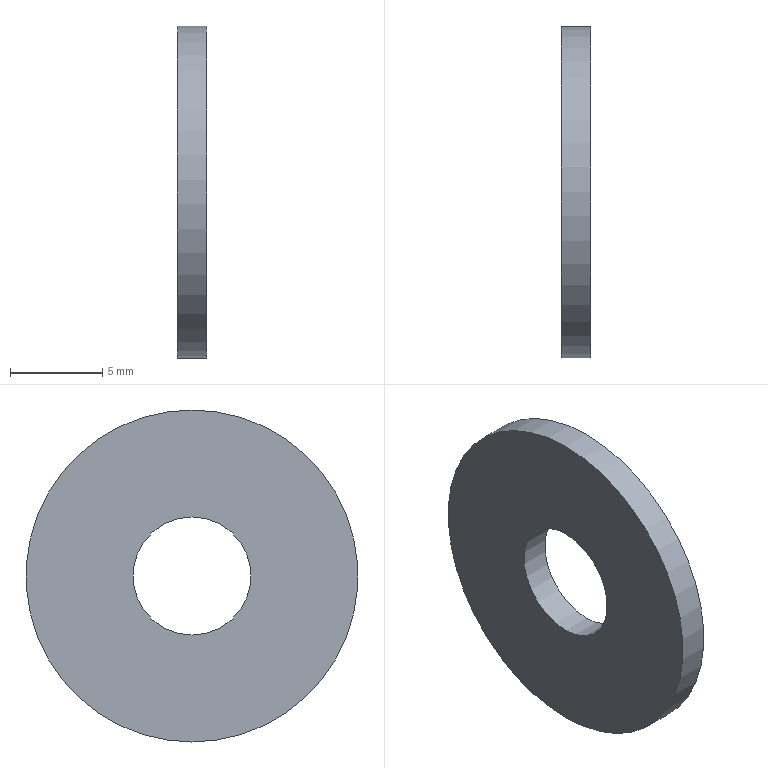Component | NX | GB-T96_1-2002_M6 | 1 solid | 4 faces | box 1.6 x 18 x 18 mm | volume 356 mm3 | cylinder 2 | plane 2 | commonest cylinder face diameters 18 x1 6.4 x1
STEP:
#1=CARTESIAN_POINT('',(0.,0.,0.));
#2=DIRECTION('',(0.,0.,1.));
#3=DIRECTION('',(1.,0.,0.));
#4=AXIS2_PLACEMENT_3D('',#1,#2,#3);
#5=CARTESIAN_POINT('',(6.,-32.,-48.));
#6=VERTEX_POINT('',#5);
#7=CARTESIAN_POINT('',(6.,-32.,-57.));
#8=DIRECTION('',(1.,0.,0.));
#9=DIRECTION('',(0.,0.,1.));
#10=AXIS2_PLACEMENT_3D('',#7,#8,#9);
#11=CIRCLE('',#10,9.);
#12=CARTESIAN_POINT('',(6.,-32.,-57.));
#13=DIRECTION('',(-1.,0.,0.));
#14=DIRECTION('',(0.,0.,-1.));
#15=AXIS2_PLACEMENT_3D('',#12,#13,#14);
#16=CYLINDRICAL_SURFACE('',#15,9.);
#17=CARTESIAN_POINT('',(9.425,0.));
#18=DIRECTION('',(-1.,0.));
#19=VECTOR('',#18,1.);
#20=LINE('',#17,#19);
#21=(GEOMETRIC_REPRESENTATION_CONTEXT(2)PARAMETRIC_REPRESENTATION_CONTEXT()REPRESENTATION_CONTEXT('',''));
#22=DEFINITIONAL_REPRESENTATION('',(#20),#21);
#23=PCURVE('',#16,#22);
#24=CARTESIAN_POINT('',(6.,-32.,-57.));
#25=DIRECTION('',(1.,0.,0.));
#26=DIRECTION('',(0.,0.,1.));
#27=AXIS2_PLACEMENT_3D('',#24,#25,#26);
#28=PLANE('',#27);
#29=CARTESIAN_POINT('',(0.,0.));
#30=DIRECTION('',(1.,0.));
#31=AXIS2_PLACEMENT_2D('',#29,#30);
#32=CIRCLE('',#31,9.);
#33=(GEOMETRIC_REPRESENTATION_CONTEXT(2)PARAMETRIC_REPRESENTATION_CONTEXT()REPRESENTATION_CONTEXT('',''));
#34=DEFINITIONAL_REPRESENTATION('',(#32),#33);
#35=PCURVE('',#28,#34);
#36=SURFACE_CURVE('',#11,(#23,#35),.PCURVE_S1.);
#37=EDGE_CURVE('',#6,#6,#36,.T.);
#38=ORIENTED_EDGE('',*,*,#37,.F.);
#39=CARTESIAN_POINT('',(4.4,-32.,-48.));
#40=VERTEX_POINT('',#39);
#41=CARTESIAN_POINT('',(6.,-32.,-48.));
#42=CARTESIAN_POINT('',(4.4,-32.,-48.));
#43=B_SPLINE_CURVE_WITH_KNOTS('',1,(#41,#42),.UNSPECIFIED.,.F.,.F.,(2,2),(0.,1.6),.PIECEWISE_BEZIER_KNOTS.);
#44=CARTESIAN_POINT('',(9.425,0.));
#45=DIRECTION('',(0.,1.));
#46=VECTOR('',#45,1.);
#47=LINE('',#44,#46);
#48=(GEOMETRIC_REPRESENTATION_CONTEXT(2)PARAMETRIC_REPRESENTATION_CONTEXT()REPRESENTATION_CONTEXT('',''));
#49=DEFINITIONAL_REPRESENTATION('',(#47),#48);
#50=PCURVE('',#16,#49);
#51=CARTESIAN_POINT('',(3.142,0.));
#52=DIRECTION('',(0.,1.));
#53=VECTOR('',#52,1.);
#54=LINE('',#51,#53);
#55=(GEOMETRIC_REPRESENTATION_CONTEXT(2)PARAMETRIC_REPRESENTATION_CONTEXT()REPRESENTATION_CONTEXT('',''));
#56=DEFINITIONAL_REPRESENTATION('',(#54),#55);
#57=PCURVE('',#16,#56);
#58=SEAM_CURVE('',#43,(#50,#57),.PCURVE_S1.);
#59=EDGE_CURVE('',#6,#40,#58,.T.);
#60=ORIENTED_EDGE('',*,*,#59,.T.);
#61=CARTESIAN_POINT('',(4.4,-32.,-57.));
#62=DIRECTION('',(1.,0.,0.));
#63=DIRECTION('',(0.,0.,1.));
#64=AXIS2_PLACEMENT_3D('',#61,#62,#63);
#65=CIRCLE('',#64,9.);
#66=CARTESIAN_POINT('',(9.425,1.6));
#67=DIRECTION('',(-1.,0.));
#68=VECTOR('',#67,1.);
#69=LINE('',#66,#68);
#70=(GEOMETRIC_REPRESENTATION_CONTEXT(2)PARAMETRIC_REPRESENTATION_CONTEXT()REPRESENTATION_CONTEXT('',''));
#71=DEFINITIONAL_REPRESENTATION('',(#69),#70);
#72=PCURVE('',#16,#71);
#73=CARTESIAN_POINT('',(4.4,-32.,-57.));
#74=DIRECTION('',(1.,0.,0.));
#75=DIRECTION('',(0.,0.,1.));
#76=AXIS2_PLACEMENT_3D('',#73,#74,#75);
#77=PLANE('',#76);
#78=CARTESIAN_POINT('',(0.,0.));
#79=DIRECTION('',(1.,0.));
#80=AXIS2_PLACEMENT_2D('',#78,#79);
#81=CIRCLE('',#80,9.);
#82=(GEOMETRIC_REPRESENTATION_CONTEXT(2)PARAMETRIC_REPRESENTATION_CONTEXT()REPRESENTATION_CONTEXT('',''));
#83=DEFINITIONAL_REPRESENTATION('',(#81),#82);
#84=PCURVE('',#77,#83);
#85=SURFACE_CURVE('',#65,(#72,#84),.PCURVE_S1.);
#86=EDGE_CURVE('',#40,#40,#85,.T.);
#87=ORIENTED_EDGE('',*,*,#86,.T.);
#88=ORIENTED_EDGE('',*,*,#59,.F.);
#89=EDGE_LOOP('',(#38,#60,#87,#88));
#90=FACE_BOUND('',#89,.T.);
#91=ADVANCED_FACE('',(#90),#16,.T.);
#92=CARTESIAN_POINT('',(6.,-32.,-53.8));
#93=VERTEX_POINT('',#92);
#94=CARTESIAN_POINT('',(6.,-32.,-57.));
#95=DIRECTION('',(1.,0.,0.));
#96=DIRECTION('',(0.,0.,1.));
#97=AXIS2_PLACEMENT_3D('',#94,#95,#96);
#98=CIRCLE('',#97,3.2);
#99=CARTESIAN_POINT('',(6.,-32.,-57.));
#100=DIRECTION('',(-1.,0.,0.));
#101=DIRECTION('',(0.,0.,-1.));
#102=AXIS2_PLACEMENT_3D('',#99,#100,#101);
#103=CYLINDRICAL_SURFACE('',#102,3.2);
#104=CARTESIAN_POINT('',(9.425,0.));
#105=DIRECTION('',(-1.,0.));
#106=VECTOR('',#105,1.);
#107=LINE('',#104,#106);
#108=(GEOMETRIC_REPRESENTATION_CONTEXT(2)PARAMETRIC_REPRESENTATION_CONTEXT()REPRESENTATION_CONTEXT('',''));
#109=DEFINITIONAL_REPRESENTATION('',(#107),#108);
#110=PCURVE('',#103,#109);
#111=CARTESIAN_POINT('',(0.,0.));
#112=DIRECTION('',(1.,0.));
#113=AXIS2_PLACEMENT_2D('',#111,#112);
#114=CIRCLE('',#113,3.2);
#115=(GEOMETRIC_REPRESENTATION_CONTEXT(2)PARAMETRIC_REPRESENTATION_CONTEXT()REPRESENTATION_CONTEXT('',''));
#116=DEFINITIONAL_REPRESENTATION('',(#114),#115);
#117=PCURVE('',#28,#116);
#118=SURFACE_CURVE('',#98,(#110,#117),.PCURVE_S1.);
#119=EDGE_CURVE('',#93,#93,#118,.T.);
#120=ORIENTED_EDGE('',*,*,#119,.F.);
#121=CARTESIAN_POINT('',(4.4,-32.,-53.8));
#122=VERTEX_POINT('',#121);
#123=CARTESIAN_POINT('',(6.,-32.,-53.8));
#124=CARTESIAN_POINT('',(4.4,-32.,-53.8));
#125=B_SPLINE_CURVE_WITH_KNOTS('',1,(#123,#124),.UNSPECIFIED.,.F.,.F.,(2,2),(0.,1.6),.PIECEWISE_BEZIER_KNOTS.);
#126=CARTESIAN_POINT('',(9.425,0.));
#127=DIRECTION('',(0.,1.));
#128=VECTOR('',#127,1.);
#129=LINE('',#126,#128);
#130=(GEOMETRIC_REPRESENTATION_CONTEXT(2)PARAMETRIC_REPRESENTATION_CONTEXT()REPRESENTATION_CONTEXT('',''));
#131=DEFINITIONAL_REPRESENTATION('',(#129),#130);
#132=PCURVE('',#103,#131);
#133=CARTESIAN_POINT('',(3.142,0.));
#134=DIRECTION('',(0.,1.));
#135=VECTOR('',#134,1.);
#136=LINE('',#133,#135);
#137=(GEOMETRIC_REPRESENTATION_CONTEXT(2)PARAMETRIC_REPRESENTATION_CONTEXT()REPRESENTATION_CONTEXT('',''));
#138=DEFINITIONAL_REPRESENTATION('',(#136),#137);
#139=PCURVE('',#103,#138);
#140=SEAM_CURVE('',#125,(#132,#139),.PCURVE_S1.);
#141=EDGE_CURVE('',#93,#122,#140,.T.);
#142=ORIENTED_EDGE('',*,*,#141,.T.);
#143=CARTESIAN_POINT('',(4.4,-32.,-57.));
#144=DIRECTION('',(1.,0.,0.));
#145=DIRECTION('',(0.,0.,1.));
#146=AXIS2_PLACEMENT_3D('',#143,#144,#145);
#147=CIRCLE('',#146,3.2);
#148=CARTESIAN_POINT('',(9.425,1.6));
#149=DIRECTION('',(-1.,0.));
#150=VECTOR('',#149,1.);
#151=LINE('',#148,#150);
#152=(GEOMETRIC_REPRESENTATION_CONTEXT(2)PARAMETRIC_REPRESENTATION_CONTEXT()REPRESENTATION_CONTEXT('',''));
#153=DEFINITIONAL_REPRESENTATION('',(#151),#152);
#154=PCURVE('',#103,#153);
#155=CARTESIAN_POINT('',(0.,0.));
#156=DIRECTION('',(1.,0.));
#157=AXIS2_PLACEMENT_2D('',#155,#156);
#158=CIRCLE('',#157,3.2);
#159=(GEOMETRIC_REPRESENTATION_CONTEXT(2)PARAMETRIC_REPRESENTATION_CONTEXT()REPRESENTATION_CONTEXT('',''));
#160=DEFINITIONAL_REPRESENTATION('',(#158),#159);
#161=PCURVE('',#77,#160);
#162=SURFACE_CURVE('',#147,(#154,#161),.PCURVE_S1.);
#163=EDGE_CURVE('',#122,#122,#162,.T.);
#164=ORIENTED_EDGE('',*,*,#163,.T.);
#165=ORIENTED_EDGE('',*,*,#141,.F.);
#166=EDGE_LOOP('',(#120,#142,#164,#165));
#167=FACE_BOUND('',#166,.F.);
#168=ADVANCED_FACE('',(#167),#103,.F.);
#169=ORIENTED_EDGE('',*,*,#37,.T.);
#170=EDGE_LOOP('',(#169));
#171=FACE_BOUND('',#170,.T.);
#172=ORIENTED_EDGE('',*,*,#119,.F.);
#173=EDGE_LOOP('',(#172));
#174=FACE_BOUND('',#173,.T.);
#175=ADVANCED_FACE('',(#171,#174),#28,.T.);
#176=ORIENTED_EDGE('',*,*,#86,.F.);
#177=EDGE_LOOP('',(#176));
#178=FACE_BOUND('',#177,.T.);
#179=ORIENTED_EDGE('',*,*,#163,.T.);
#180=EDGE_LOOP('',(#179));
#181=FACE_BOUND('',#180,.T.);
#182=ADVANCED_FACE('',(#178,#181),#77,.F.);
#183=CLOSED_SHELL('',(#91,#168,#175,#182));
#184=MANIFOLD_SOLID_BREP('',#183);
#185=(LENGTH_UNIT()NAMED_UNIT(*)SI_UNIT(.MILLI.,.METRE.));
#186=UNCERTAINTY_MEASURE_WITH_UNIT(LENGTH_MEASURE(0.00001),#185,'','');
#187=(NAMED_UNIT(*)PLANE_ANGLE_UNIT()SI_UNIT($,.RADIAN.));
#188=(NAMED_UNIT(*)SI_UNIT($,.STERADIAN.)SOLID_ANGLE_UNIT());
#189=(GEOMETRIC_REPRESENTATION_CONTEXT(3)GLOBAL_UNCERTAINTY_ASSIGNED_CONTEXT((#186))GLOBAL_UNIT_ASSIGNED_CONTEXT((#185,#187,#188))REPRESENTATION_CONTEXT('',''));
#190=ADVANCED_BREP_SHAPE_REPRESENTATION('',(#4,#184),#189);